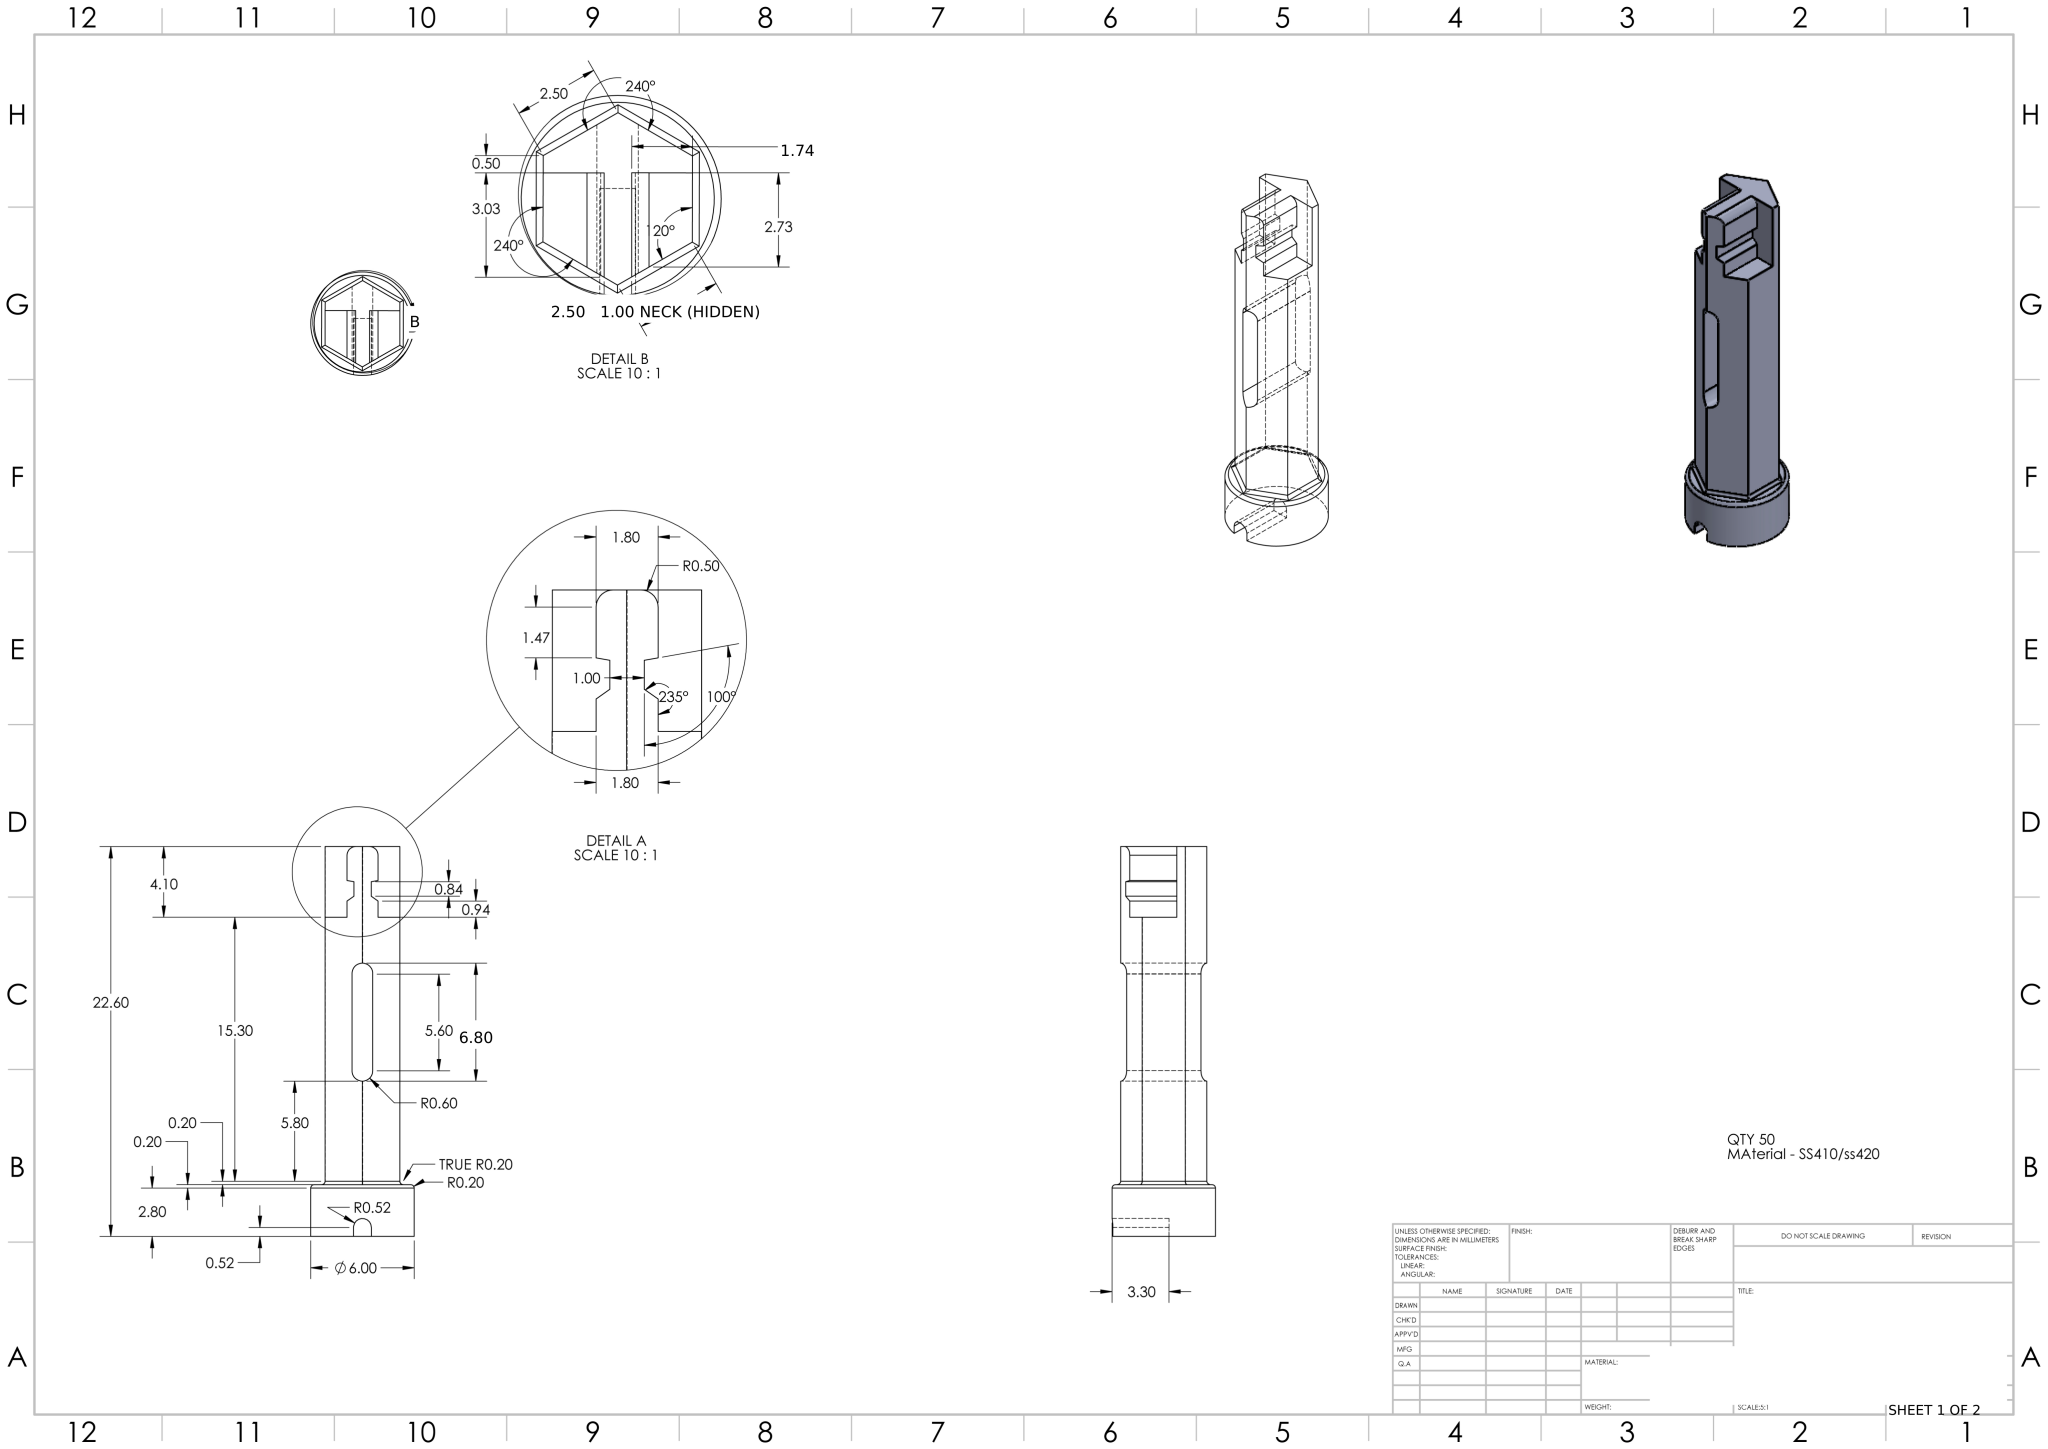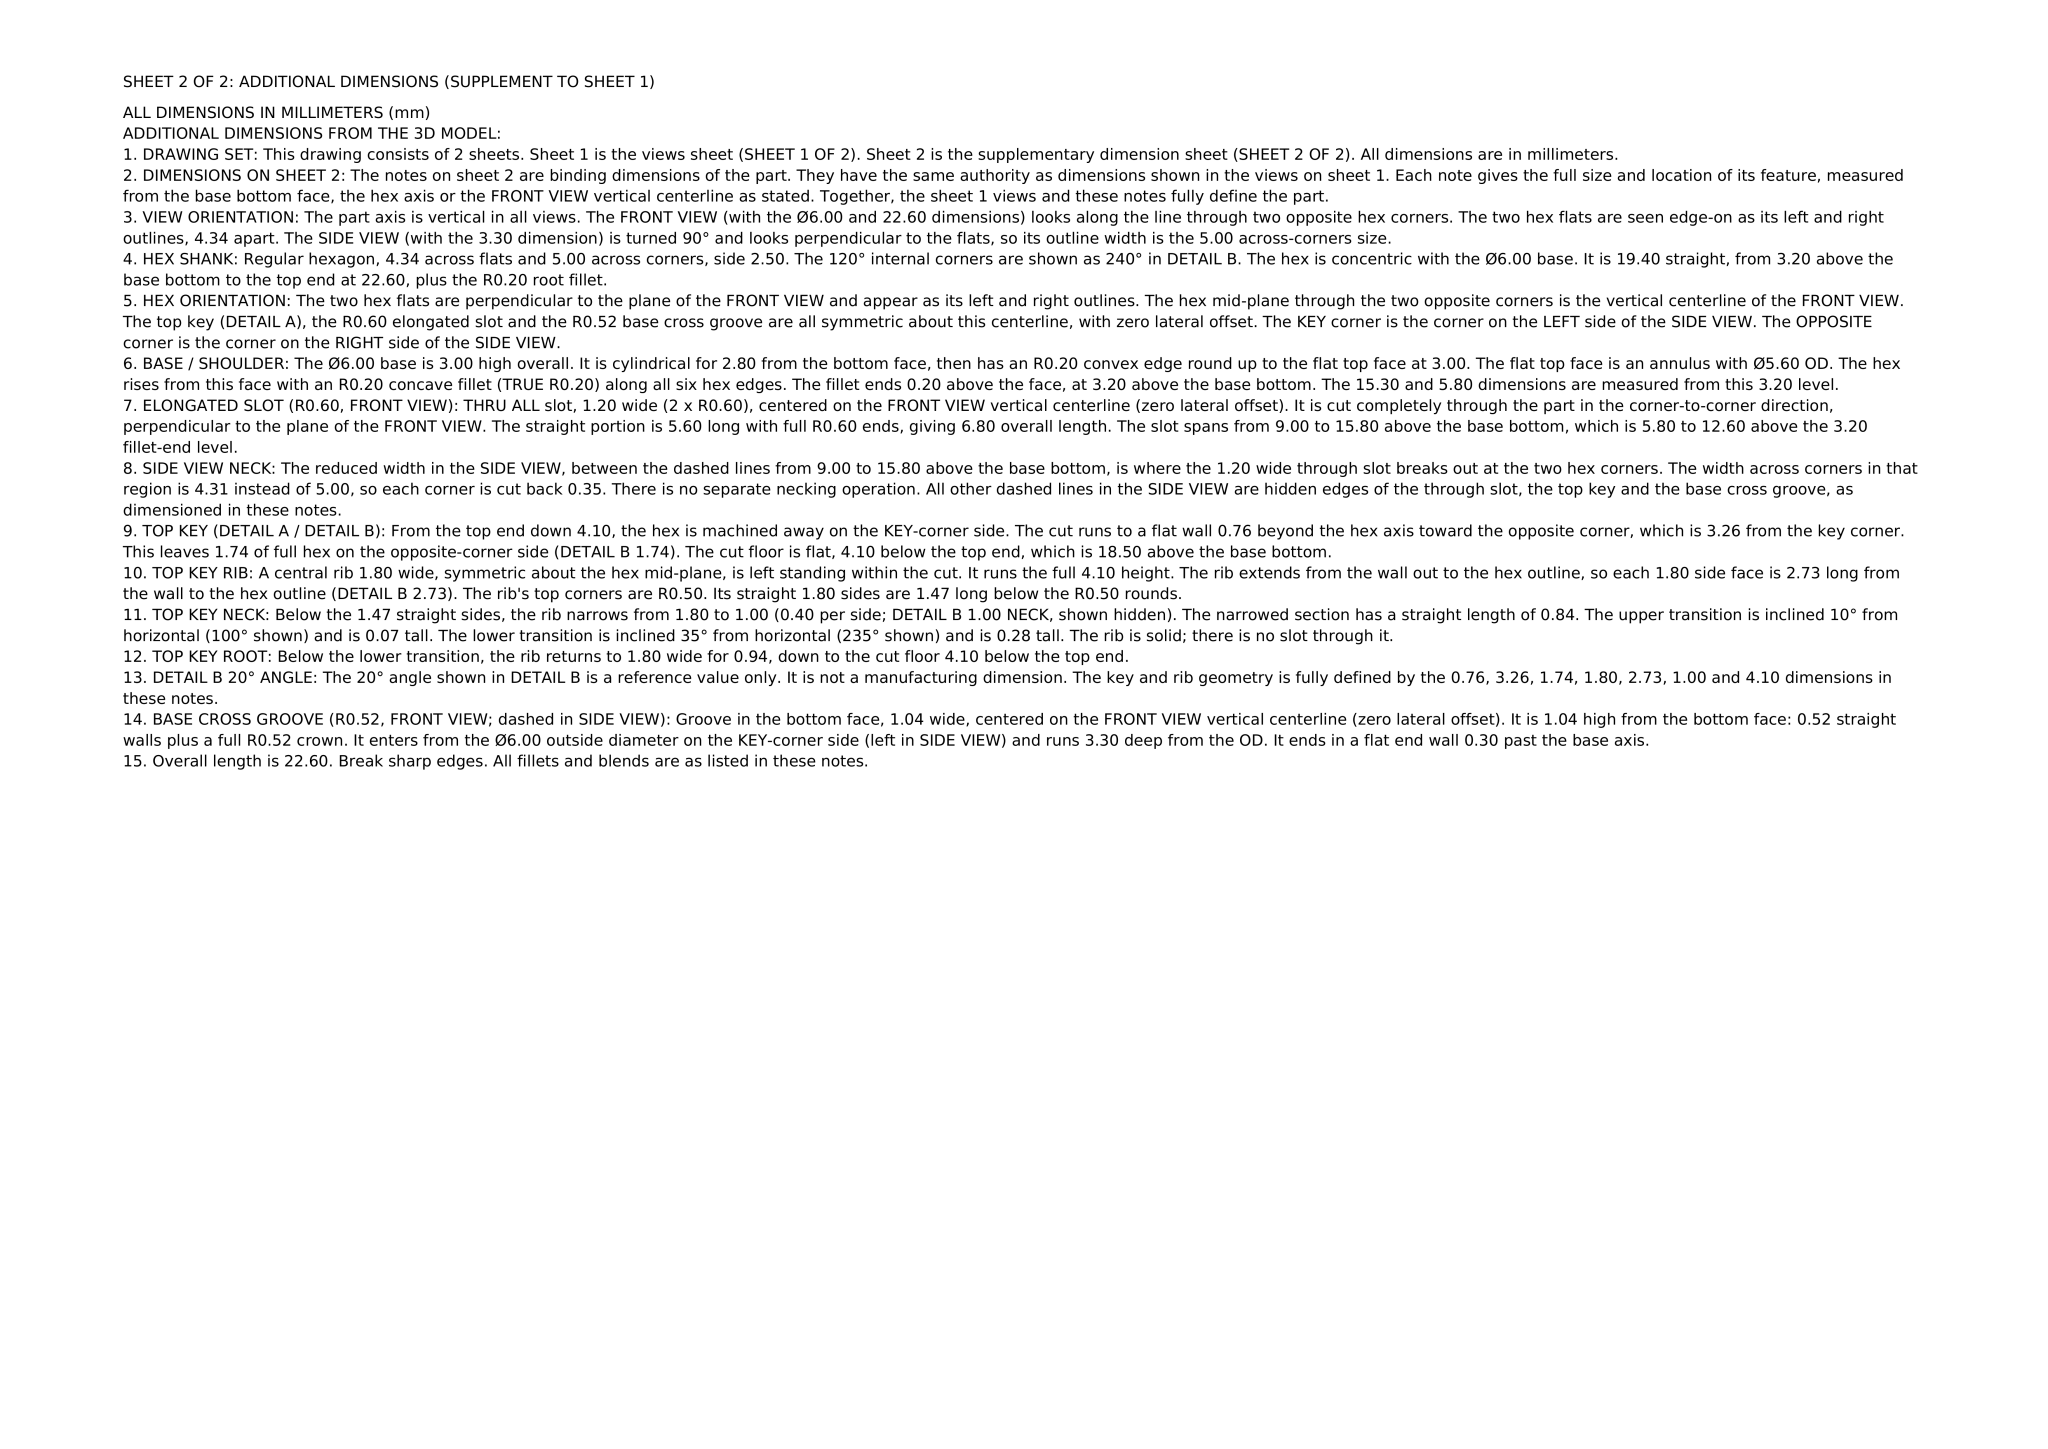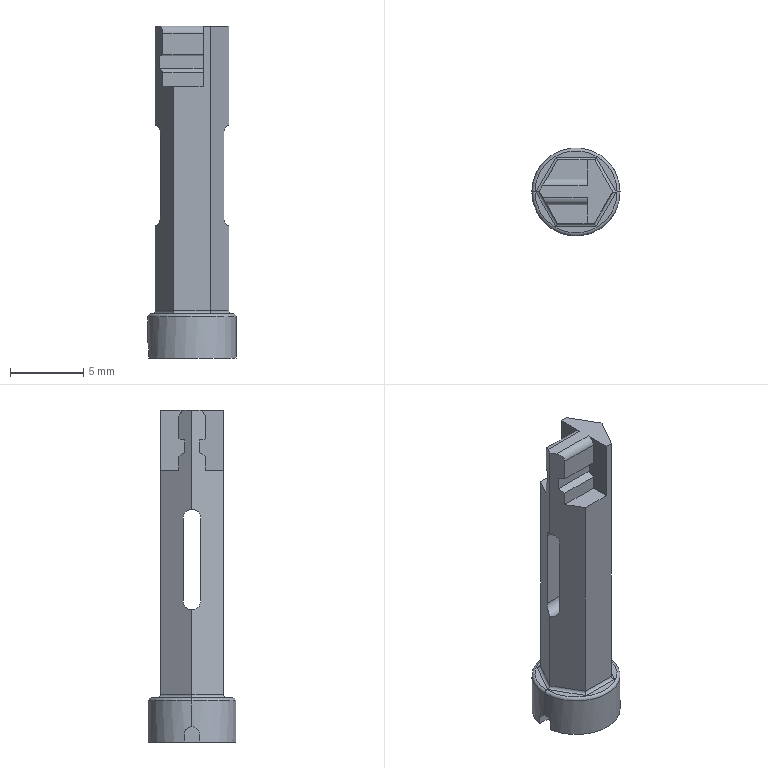Part | NX | mm | 1 solid | 48 faces | box 6 x 6 x 22.6 mm | volume 336 mm3 | plane 30 | cylinder 16 | torus 2 | commonest cylinder face diameters 0.4 x8 1.2 x3 6 x2 1 x2 1.04 x1